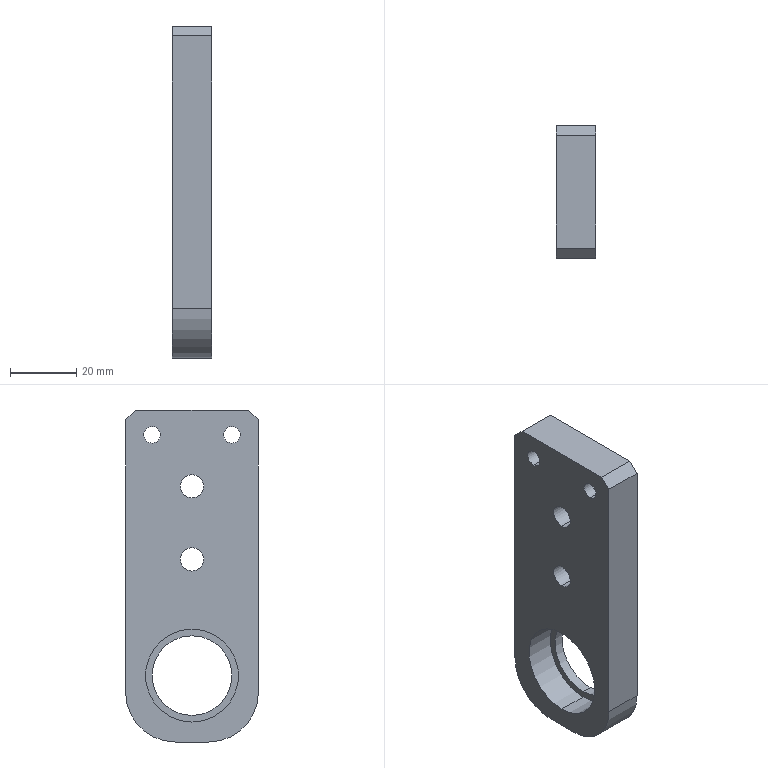Component | SolidWorks | ConveyorDrivenWheelSidePlate-4 | 1 solid | 23 faces | box 12 x 40 x 100 mm | volume 38439 mm3 | cylinder 14 | plane 9 | commonest cylinder face diameters 5 x4 7 x4 24 x2 28 x2 30 x2 | material Plain Carbon Steel
build123d program:
from build123d import *

# Parameters (mm, degrees)
SKETCH1_W           = 100
SKETCH1_H           = 40
BOSS_EXTRUDE1_DEPTH = 12
SKETCH2_R           = 14
CUT_EXTRUDE1_DEPTH  = 9
SKETCH3_R           = 3.5
CUT_EXTRUDE2_DEPTH  = 56.172
SKETCH4_R           = 12
CUT_EXTRUDE3_DEPTH  = 55.599
FILLET1_R           = 15
CHAMFER1_SIZE       = 3
M6_TAPPED_HOLE1_D   = 5


with BuildPart() as part:
    # Sketch1 → Boss-Extrude1 (new body)
    with BuildSketch(Plane(origin=(0, 0, 0), x_dir=(0, 0, -1), z_dir=(1, 0, 0))):
        Rectangle(SKETCH1_W, SKETCH1_H)
    extrude(amount=BOSS_EXTRUDE1_DEPTH)

    # Sketch2 → Cut-Extrude1 (cut)
    with BuildSketch(Plane(origin=(12, 0, 0), x_dir=(0, 0, -1), z_dir=(1, 0, 0))):
        with Locations((30, 0)):
            Circle(SKETCH2_R)
    extrude(amount=-CUT_EXTRUDE1_DEPTH, mode=Mode.SUBTRACT)

    # Sketch3 → Cut-Extrude2 (cut, through all)
    with BuildSketch(Plane.ZY):
        with Locations((5, 0)):
            Circle(SKETCH3_R)
        with Locations((27, 0)):
            Circle(SKETCH3_R)
    extrude(amount=-CUT_EXTRUDE2_DEPTH, mode=Mode.SUBTRACT)

    # Sketch4 → Cut-Extrude3 (cut, through all)
    with BuildSketch(Plane(origin=(3, 0, 0), x_dir=(0, 0, -1), z_dir=(1, 0, 0))):
        with Locations((30, 0)):
            Circle(SKETCH4_R)
    extrude(amount=-CUT_EXTRUDE3_DEPTH, mode=Mode.SUBTRACT)

    # Fillet1
    fillet1_edges = [part.edges().sort_by_distance(p)[0] for p in [
        (6, -20, -50),
        (6, 20, -50),
    ]]
    fillet(fillet1_edges, radius=FILLET1_R)

    # Chamfer1
    chamfer1_edges = [part.edges().sort_by_distance(p)[0] for p in [
        (6, -20, 50),
        (6, 20, 50),
    ]]
    chamfer(chamfer1_edges, length=CHAMFER1_SIZE)

    # M6 Tapped Hole1 (through all)
    with Locations(Plane.ZY):
        with Locations((42.5, 12), (42.5, -12)):
            Hole(M6_TAPPED_HOLE1_D / 2)


solid = part.part

# Placed as in the assembly
solid = solid.moved(Location((47.45, 5.646, 185), (0, 0, 180)))
STEP:
#1=COLOUR_RGB('',0.7922,0.8196,0.9333);
#2=FILL_AREA_STYLE_COLOUR('',#1);
#3=FILL_AREA_STYLE('',(#2));
#4=SURFACE_STYLE_FILL_AREA(#3);
#5=SURFACE_SIDE_STYLE('',(#4));
#6=SURFACE_STYLE_USAGE(.BOTH.,#5);
#7=PRESENTATION_STYLE_ASSIGNMENT((#6));
#8=CARTESIAN_POINT('',(1.396,-0.2502,8.858));
#9=VERTEX_POINT('',#8);
#10=CARTESIAN_POINT('',(1.396,-0.2502,9.055));
#11=VERTEX_POINT('',#10);
#12=CARTESIAN_POINT('',(1.396,-0.2502,8.957));
#13=DIRECTION('',(1.,-0.,-0.));
#14=DIRECTION('',(0.,0.,1.));
#15=AXIS2_PLACEMENT_3D('',#12,#13,#14);
#16=CIRCLE('',#15,0.09843);
#17=EDGE_CURVE('',#9,#11,#16,.T.);
#18=ORIENTED_EDGE('',*,*,#17,.F.);
#19=CARTESIAN_POINT('',(1.868,-0.2502,8.858));
#20=VERTEX_POINT('',#19);
#21=CARTESIAN_POINT('',(1.868,-0.2502,8.858));
#22=DIRECTION('',(1.,-0.,-0.));
#23=VECTOR('',#22,39.37);
#24=LINE('',#21,#23);
#25=EDGE_CURVE('',#9,#20,#24,.T.);
#26=ORIENTED_EDGE('',*,*,#25,.T.);
#27=CARTESIAN_POINT('',(1.868,-0.2502,9.055));
#28=VERTEX_POINT('',#27);
#29=CARTESIAN_POINT('',(1.868,-0.2502,8.957));
#30=DIRECTION('',(1.,-0.,-0.));
#31=DIRECTION('',(0.,0.,1.));
#32=AXIS2_PLACEMENT_3D('',#29,#30,#31);
#33=CIRCLE('',#32,0.09843);
#34=EDGE_CURVE('',#20,#28,#33,.T.);
#35=ORIENTED_EDGE('',*,*,#34,.T.);
#36=CARTESIAN_POINT('',(1.868,-0.2502,9.055));
#37=DIRECTION('',(1.,-0.,-0.));
#38=VECTOR('',#37,39.37);
#39=LINE('',#36,#38);
#40=EDGE_CURVE('',#11,#28,#39,.T.);
#41=ORIENTED_EDGE('',*,*,#40,.F.);
#42=EDGE_LOOP('',(#18,#26,#35,#41));
#43=FACE_OUTER_BOUND('',#42,.T.);
#44=CARTESIAN_POINT('',(1.868,-0.2502,8.957));
#45=DIRECTION('',(1.,-0.,-0.));
#46=DIRECTION('',(0.,0.,1.));
#47=AXIS2_PLACEMENT_3D('',#44,#45,#46);
#48=CYLINDRICAL_SURFACE('',#47,0.09843);
#49=ADVANCED_FACE('',(#43),#48,.F.);
#50=CARTESIAN_POINT('',(1.396,0.6947,8.858));
#51=VERTEX_POINT('',#50);
#52=CARTESIAN_POINT('',(1.396,0.6947,9.055));
#53=VERTEX_POINT('',#52);
#54=CARTESIAN_POINT('',(1.396,0.6947,8.957));
#55=DIRECTION('',(1.,-0.,-0.));
#56=DIRECTION('',(0.,0.,1.));
#57=AXIS2_PLACEMENT_3D('',#54,#55,#56);
#58=CIRCLE('',#57,0.09843);
#59=EDGE_CURVE('',#51,#53,#58,.T.);
#60=ORIENTED_EDGE('',*,*,#59,.F.);
#61=CARTESIAN_POINT('',(1.868,0.6947,8.858));
#62=VERTEX_POINT('',#61);
#63=CARTESIAN_POINT('',(1.868,0.6947,8.858));
#64=DIRECTION('',(1.,-0.,-0.));
#65=VECTOR('',#64,39.37);
#66=LINE('',#63,#65);
#67=EDGE_CURVE('',#51,#62,#66,.T.);
#68=ORIENTED_EDGE('',*,*,#67,.T.);
#69=CARTESIAN_POINT('',(1.868,0.6947,9.055));
#70=VERTEX_POINT('',#69);
#71=CARTESIAN_POINT('',(1.868,0.6947,8.957));
#72=DIRECTION('',(1.,-0.,-0.));
#73=DIRECTION('',(0.,0.,1.));
#74=AXIS2_PLACEMENT_3D('',#71,#72,#73);
#75=CIRCLE('',#74,0.09843);
#76=EDGE_CURVE('',#62,#70,#75,.T.);
#77=ORIENTED_EDGE('',*,*,#76,.T.);
#78=CARTESIAN_POINT('',(1.868,0.6947,9.055));
#79=DIRECTION('',(1.,-0.,-0.));
#80=VECTOR('',#79,39.37);
#81=LINE('',#78,#80);
#82=EDGE_CURVE('',#53,#70,#81,.T.);
#83=ORIENTED_EDGE('',*,*,#82,.F.);
#84=EDGE_LOOP('',(#60,#68,#77,#83));
#85=FACE_OUTER_BOUND('',#84,.T.);
#86=CARTESIAN_POINT('',(1.868,0.6947,8.957));
#87=DIRECTION('',(1.,-0.,-0.));
#88=DIRECTION('',(0.,0.,1.));
#89=AXIS2_PLACEMENT_3D('',#86,#87,#88);
#90=CYLINDRICAL_SURFACE('',#89,0.09843);
#91=ADVANCED_FACE('',(#85),#90,.F.);
#92=CARTESIAN_POINT('',(1.868,0.2223,6.575));
#93=VERTEX_POINT('',#92);
#94=CARTESIAN_POINT('',(1.868,0.2223,5.63));
#95=VERTEX_POINT('',#94);
#96=CARTESIAN_POINT('',(1.868,0.2223,6.102));
#97=DIRECTION('',(-1.,0.,0.));
#98=DIRECTION('',(0.,0.,-1.));
#99=AXIS2_PLACEMENT_3D('',#96,#97,#98);
#100=CIRCLE('',#99,0.4724);
#101=EDGE_CURVE('',#93,#95,#100,.T.);
#102=ORIENTED_EDGE('',*,*,#101,.F.);
#103=CARTESIAN_POINT('',(1.75,0.2223,6.575));
#104=VERTEX_POINT('',#103);
#105=CARTESIAN_POINT('',(1.868,0.2223,6.575));
#106=DIRECTION('',(-1.,0.,0.));
#107=VECTOR('',#106,39.37);
#108=LINE('',#105,#107);
#109=EDGE_CURVE('',#93,#104,#108,.T.);
#110=ORIENTED_EDGE('',*,*,#109,.T.);
#111=CARTESIAN_POINT('',(1.75,0.2223,5.63));
#112=VERTEX_POINT('',#111);
#113=CARTESIAN_POINT('',(1.75,0.2223,6.102));
#114=DIRECTION('',(-1.,0.,0.));
#115=DIRECTION('',(0.,0.,-1.));
#116=AXIS2_PLACEMENT_3D('',#113,#114,#115);
#117=CIRCLE('',#116,0.4724);
#118=EDGE_CURVE('',#104,#112,#117,.T.);
#119=ORIENTED_EDGE('',*,*,#118,.T.);
#120=CARTESIAN_POINT('',(1.868,0.2223,5.63));
#121=DIRECTION('',(-1.,0.,0.));
#122=VECTOR('',#121,39.37);
#123=LINE('',#120,#122);
#124=EDGE_CURVE('',#95,#112,#123,.T.);
#125=ORIENTED_EDGE('',*,*,#124,.F.);
#126=EDGE_LOOP('',(#102,#110,#119,#125));
#127=FACE_OUTER_BOUND('',#126,.T.);
#128=CARTESIAN_POINT('',(1.868,0.2223,6.102));
#129=DIRECTION('',(-1.,0.,0.));
#130=DIRECTION('',(0.,0.,-1.));
#131=AXIS2_PLACEMENT_3D('',#128,#129,#130);
#132=CYLINDRICAL_SURFACE('',#131,0.4724);
#133=ADVANCED_FACE('',(#127),#132,.F.);
#134=CARTESIAN_POINT('',(1.396,0.2223,8.209));
#135=VERTEX_POINT('',#134);
#136=CARTESIAN_POINT('',(1.396,0.2223,8.484));
#137=VERTEX_POINT('',#136);
#138=CARTESIAN_POINT('',(1.396,0.2223,8.346));
#139=DIRECTION('',(1.,-0.,-0.));
#140=DIRECTION('',(0.,0.,1.));
#141=AXIS2_PLACEMENT_3D('',#138,#139,#140);
#142=CIRCLE('',#141,0.1378);
#143=EDGE_CURVE('',#135,#137,#142,.T.);
#144=ORIENTED_EDGE('',*,*,#143,.F.);
#145=CARTESIAN_POINT('',(1.868,0.2223,8.209));
#146=VERTEX_POINT('',#145);
#147=CARTESIAN_POINT('',(1.396,0.2223,8.209));
#148=DIRECTION('',(1.,-0.,-0.));
#149=VECTOR('',#148,39.37);
#150=LINE('',#147,#149);
#151=EDGE_CURVE('',#135,#146,#150,.T.);
#152=ORIENTED_EDGE('',*,*,#151,.T.);
#153=CARTESIAN_POINT('',(1.868,0.2223,8.484));
#154=VERTEX_POINT('',#153);
#155=CARTESIAN_POINT('',(1.868,0.2223,8.346));
#156=DIRECTION('',(1.,-0.,-0.));
#157=DIRECTION('',(0.,0.,1.));
#158=AXIS2_PLACEMENT_3D('',#155,#156,#157);
#159=CIRCLE('',#158,0.1378);
#160=EDGE_CURVE('',#146,#154,#159,.T.);
#161=ORIENTED_EDGE('',*,*,#160,.T.);
#162=CARTESIAN_POINT('',(1.396,0.2223,8.484));
#163=DIRECTION('',(1.,-0.,-0.));
#164=VECTOR('',#163,39.37);
#165=LINE('',#162,#164);
#166=EDGE_CURVE('',#137,#154,#165,.T.);
#167=ORIENTED_EDGE('',*,*,#166,.F.);
#168=EDGE_LOOP('',(#144,#152,#161,#167));
#169=FACE_OUTER_BOUND('',#168,.T.);
#170=CARTESIAN_POINT('',(1.396,0.2223,8.346));
#171=DIRECTION('',(1.,-0.,-0.));
#172=DIRECTION('',(0.,0.,1.));
#173=AXIS2_PLACEMENT_3D('',#170,#171,#172);
#174=CYLINDRICAL_SURFACE('',#173,0.1378);
#175=ADVANCED_FACE('',(#169),#174,.F.);
#176=CARTESIAN_POINT('',(1.396,0.2223,7.343));
#177=VERTEX_POINT('',#176);
#178=CARTESIAN_POINT('',(1.396,0.2223,7.618));
#179=VERTEX_POINT('',#178);
#180=CARTESIAN_POINT('',(1.396,0.2223,7.48));
#181=DIRECTION('',(1.,-0.,-0.));
#182=DIRECTION('',(0.,0.,1.));
#183=AXIS2_PLACEMENT_3D('',#180,#181,#182);
#184=CIRCLE('',#183,0.1378);
#185=EDGE_CURVE('',#177,#179,#184,.T.);
#186=ORIENTED_EDGE('',*,*,#185,.F.);
#187=CARTESIAN_POINT('',(1.868,0.2223,7.343));
#188=VERTEX_POINT('',#187);
#189=CARTESIAN_POINT('',(1.396,0.2223,7.343));
#190=DIRECTION('',(1.,-0.,-0.));
#191=VECTOR('',#190,39.37);
#192=LINE('',#189,#191);
#193=EDGE_CURVE('',#177,#188,#192,.T.);
#194=ORIENTED_EDGE('',*,*,#193,.T.);
#195=CARTESIAN_POINT('',(1.868,0.2223,7.618));
#196=VERTEX_POINT('',#195);
#197=CARTESIAN_POINT('',(1.868,0.2223,7.48));
#198=DIRECTION('',(1.,-0.,-0.));
#199=DIRECTION('',(0.,0.,1.));
#200=AXIS2_PLACEMENT_3D('',#197,#198,#199);
#201=CIRCLE('',#200,0.1378);
#202=EDGE_CURVE('',#188,#196,#201,.T.);
#203=ORIENTED_EDGE('',*,*,#202,.T.);
#204=CARTESIAN_POINT('',(1.396,0.2223,7.618));
#205=DIRECTION('',(1.,-0.,-0.));
#206=VECTOR('',#205,39.37);
#207=LINE('',#204,#206);
#208=EDGE_CURVE('',#179,#196,#207,.T.);
#209=ORIENTED_EDGE('',*,*,#208,.F.);
#210=EDGE_LOOP('',(#186,#194,#203,#209));
#211=FACE_OUTER_BOUND('',#210,.T.);
#212=CARTESIAN_POINT('',(1.396,0.2223,7.48));
#213=DIRECTION('',(1.,-0.,-0.));
#214=DIRECTION('',(0.,0.,1.));
#215=AXIS2_PLACEMENT_3D('',#212,#213,#214);
#216=CYLINDRICAL_SURFACE('',#215,0.1378);
#217=ADVANCED_FACE('',(#211),#216,.F.);
#218=CARTESIAN_POINT('',(1.75,0.2223,6.654));
#219=VERTEX_POINT('',#218);
#220=CARTESIAN_POINT('',(1.75,0.2223,5.551));
#221=VERTEX_POINT('',#220);
#222=CARTESIAN_POINT('',(1.75,0.2223,6.102));
#223=DIRECTION('',(-1.,0.,0.));
#224=DIRECTION('',(0.,0.,-1.));
#225=AXIS2_PLACEMENT_3D('',#222,#223,#224);
#226=CIRCLE('',#225,0.5512);
#227=EDGE_CURVE('',#219,#221,#226,.T.);
#228=ORIENTED_EDGE('',*,*,#227,.F.);
#229=CARTESIAN_POINT('',(1.396,0.2223,6.654));
#230=VERTEX_POINT('',#229);
#231=CARTESIAN_POINT('',(1.75,0.2223,6.654));
#232=DIRECTION('',(-1.,0.,0.));
#233=VECTOR('',#232,39.37);
#234=LINE('',#231,#233);
#235=EDGE_CURVE('',#219,#230,#234,.T.);
#236=ORIENTED_EDGE('',*,*,#235,.T.);
#237=CARTESIAN_POINT('',(1.396,0.2223,5.551));
#238=VERTEX_POINT('',#237);
#239=CARTESIAN_POINT('',(1.396,0.2223,6.102));
#240=DIRECTION('',(-1.,0.,0.));
#241=DIRECTION('',(0.,0.,-1.));
#242=AXIS2_PLACEMENT_3D('',#239,#240,#241);
#243=CIRCLE('',#242,0.5512);
#244=EDGE_CURVE('',#230,#238,#243,.T.);
#245=ORIENTED_EDGE('',*,*,#244,.T.);
#246=CARTESIAN_POINT('',(1.75,0.2223,5.551));
#247=DIRECTION('',(-1.,0.,0.));
#248=VECTOR('',#247,39.37);
#249=LINE('',#246,#248);
#250=EDGE_CURVE('',#221,#238,#249,.T.);
#251=ORIENTED_EDGE('',*,*,#250,.F.);
#252=EDGE_LOOP('',(#228,#236,#245,#251));
#253=FACE_OUTER_BOUND('',#252,.T.);
#254=CARTESIAN_POINT('',(1.75,0.2223,6.102));
#255=DIRECTION('',(-1.,0.,0.));
#256=DIRECTION('',(0.,0.,-1.));
#257=AXIS2_PLACEMENT_3D('',#254,#255,#256);
#258=CYLINDRICAL_SURFACE('',#257,0.5512);
#259=ADVANCED_FACE('',(#253),#258,.F.);
#260=CARTESIAN_POINT('',(1.396,0.4191,5.315));
#261=VERTEX_POINT('',#260);
#262=CARTESIAN_POINT('',(1.396,0.02542,5.315));
#263=VERTEX_POINT('',#262);
#264=CARTESIAN_POINT('',(1.396,1.01,5.315));
#265=DIRECTION('',(-0.,-1.,0.));
#266=VECTOR('',#265,39.37);
#267=LINE('',#264,#266);
#268=EDGE_CURVE('',#261,#263,#267,.T.);
#269=ORIENTED_EDGE('',*,*,#268,.F.);
#270=CARTESIAN_POINT('',(1.868,0.4191,5.315));
#271=VERTEX_POINT('',#270);
#272=CARTESIAN_POINT('',(1.396,0.4191,5.315));
#273=DIRECTION('',(1.,-0.,-0.));
#274=VECTOR('',#273,39.37);
#275=LINE('',#272,#274);
#276=EDGE_CURVE('',#261,#271,#275,.T.);
#277=ORIENTED_EDGE('',*,*,#276,.T.);
#278=CARTESIAN_POINT('',(1.868,0.02542,5.315));
#279=VERTEX_POINT('',#278);
#280=CARTESIAN_POINT('',(1.868,1.01,5.315));
#281=DIRECTION('',(-0.,-1.,0.));
#282=VECTOR('',#281,39.37);
#283=LINE('',#280,#282);
#284=EDGE_CURVE('',#271,#279,#283,.T.);
#285=ORIENTED_EDGE('',*,*,#284,.T.);
#286=CARTESIAN_POINT('',(1.396,0.02542,5.315));
#287=DIRECTION('',(-1.,0.,0.));
#288=VECTOR('',#287,39.37);
#289=LINE('',#286,#288);
#290=EDGE_CURVE('',#279,#263,#289,.T.);
#291=ORIENTED_EDGE('',*,*,#290,.T.);
#292=EDGE_LOOP('',(#269,#277,#285,#291));
#293=FACE_OUTER_BOUND('',#292,.T.);
#294=CARTESIAN_POINT('',(1.396,1.01,5.315));
#295=DIRECTION('',(0.,-0.,1.));
#296=DIRECTION('',(-1.,0.,0.));
#297=AXIS2_PLACEMENT_3D('',#294,#295,#296);
#298=PLANE('',#297);
#299=ADVANCED_FACE('',(#293),#298,.F.);
#300=CARTESIAN_POINT('',(1.868,-0.5651,5.906));
#301=VERTEX_POINT('',#300);
#302=CARTESIAN_POINT('',(1.868,-0.5651,9.134));
#303=VERTEX_POINT('',#302);
#304=CARTESIAN_POINT('',(1.868,-0.5651,9.252));
#305=DIRECTION('',(0.,0.,1.));
#306=VECTOR('',#305,39.37);
#307=LINE('',#304,#306);
#308=EDGE_CURVE('',#301,#303,#307,.T.);
#309=ORIENTED_EDGE('',*,*,#308,.T.);
#310=CARTESIAN_POINT('',(1.396,-0.5651,9.134));
#311=VERTEX_POINT('',#310);
#312=CARTESIAN_POINT('',(1.396,-0.5651,9.134));
#313=DIRECTION('',(-1.,0.,0.));
#314=VECTOR('',#313,39.37);
#315=LINE('',#312,#314);
#316=EDGE_CURVE('',#303,#311,#315,.T.);
#317=ORIENTED_EDGE('',*,*,#316,.T.);
#318=CARTESIAN_POINT('',(1.396,-0.5651,5.906));
#319=VERTEX_POINT('',#318);
#320=CARTESIAN_POINT('',(1.396,-0.5651,9.252));
#321=DIRECTION('',(0.,0.,1.));
#322=VECTOR('',#321,39.37);
#323=LINE('',#320,#322);
#324=EDGE_CURVE('',#319,#311,#323,.T.);
#325=ORIENTED_EDGE('',*,*,#324,.F.);
#326=CARTESIAN_POINT('',(1.396,-0.5651,5.906));
#327=DIRECTION('',(1.,-0.,-0.));
#328=VECTOR('',#327,39.37);
#329=LINE('',#326,#328);
#330=EDGE_CURVE('',#319,#301,#329,.T.);
#331=ORIENTED_EDGE('',*,*,#330,.T.);
#332=EDGE_LOOP('',(#309,#317,#325,#331));
#333=FACE_OUTER_BOUND('',#332,.T.);
#334=CARTESIAN_POINT('',(1.396,-0.5651,9.252));
#335=DIRECTION('',(0.,1.,-0.));
#336=DIRECTION('',(-0.,0.,-1.));
#337=AXIS2_PLACEMENT_3D('',#334,#335,#336);
#338=PLANE('',#337);
#339=ADVANCED_FACE('',(#333),#338,.F.);
#340=CARTESIAN_POINT('',(1.868,-0.447,9.252));
#341=VERTEX_POINT('',#340);
#342=CARTESIAN_POINT('',(1.868,0.8916,9.252));
#343=VERTEX_POINT('',#342);
#344=CARTESIAN_POINT('',(1.868,1.01,9.252));
#345=DIRECTION('',(0.,1.,0.));
#346=VECTOR('',#345,39.37);
#347=LINE('',#344,#346);
#348=EDGE_CURVE('',#341,#343,#347,.T.);
#349=ORIENTED_EDGE('',*,*,#348,.T.);
#350=CARTESIAN_POINT('',(1.396,0.8916,9.252));
#351=VERTEX_POINT('',#350);
#352=CARTESIAN_POINT('',(1.396,0.8916,9.252));
#353=DIRECTION('',(-1.,0.,0.));
#354=VECTOR('',#353,39.37);
#355=LINE('',#352,#354);
#356=EDGE_CURVE('',#343,#351,#355,.T.);
#357=ORIENTED_EDGE('',*,*,#356,.T.);
#358=CARTESIAN_POINT('',(1.396,-0.447,9.252));
#359=VERTEX_POINT('',#358);
#360=CARTESIAN_POINT('',(1.396,1.01,9.252));
#361=DIRECTION('',(0.,1.,0.));
#362=VECTOR('',#361,39.37);
#363=LINE('',#360,#362);
#364=EDGE_CURVE('',#359,#351,#363,.T.);
#365=ORIENTED_EDGE('',*,*,#364,.F.);
#366=CARTESIAN_POINT('',(1.396,-0.447,9.252));
#367=DIRECTION('',(1.,-0.,-0.));
#368=VECTOR('',#367,39.37);
#369=LINE('',#366,#368);
#370=EDGE_CURVE('',#359,#341,#369,.T.);
#371=ORIENTED_EDGE('',*,*,#370,.T.);
#372=EDGE_LOOP('',(#349,#357,#365,#371));
#373=FACE_OUTER_BOUND('',#372,.T.);
#374=CARTESIAN_POINT('',(1.396,1.01,9.252));
#375=DIRECTION('',(-0.,0.,-1.));
#376=DIRECTION('',(1.,-0.,-0.));
#377=AXIS2_PLACEMENT_3D('',#374,#375,#376);
#378=PLANE('',#377);
#379=ADVANCED_FACE('',(#373),#378,.F.);
#380=CARTESIAN_POINT('',(1.396,1.01,9.134));
#381=VERTEX_POINT('',#380);
#382=CARTESIAN_POINT('',(1.396,1.01,5.906));
#383=VERTEX_POINT('',#382);
#384=CARTESIAN_POINT('',(1.396,1.01,9.252));
#385=DIRECTION('',(-0.,0.,-1.));
#386=VECTOR('',#385,39.37);
#387=LINE('',#384,#386);
#388=EDGE_CURVE('',#381,#383,#387,.T.);
#389=ORIENTED_EDGE('',*,*,#388,.F.);
#390=CARTESIAN_POINT('',(1.868,1.01,9.134));
#391=VERTEX_POINT('',#390);
#392=CARTESIAN_POINT('',(1.396,1.01,9.134));
#393=DIRECTION('',(1.,-0.,-0.));
#394=VECTOR('',#393,39.37);
#395=LINE('',#392,#394);
#396=EDGE_CURVE('',#381,#391,#395,.T.);
#397=ORIENTED_EDGE('',*,*,#396,.T.);
#398=CARTESIAN_POINT('',(1.868,1.01,5.906));
#399=VERTEX_POINT('',#398);
#400=CARTESIAN_POINT('',(1.868,1.01,9.252));
#401=DIRECTION('',(-0.,0.,-1.));
#402=VECTOR('',#401,39.37);
#403=LINE('',#400,#402);
#404=EDGE_CURVE('',#391,#399,#403,.T.);
#405=ORIENTED_EDGE('',*,*,#404,.T.);
#406=CARTESIAN_POINT('',(1.396,1.01,5.906));
#407=DIRECTION('',(-1.,0.,0.));
#408=VECTOR('',#407,39.37);
#409=LINE('',#406,#408);
#410=EDGE_CURVE('',#399,#383,#409,.T.);
#411=ORIENTED_EDGE('',*,*,#410,.T.);
#412=EDGE_LOOP('',(#389,#397,#405,#411));
#413=FACE_OUTER_BOUND('',#412,.T.);
#414=CARTESIAN_POINT('',(1.396,1.01,9.252));
#415=DIRECTION('',(-0.,-1.,0.));
#416=DIRECTION('',(0.,0.,1.));
#417=AXIS2_PLACEMENT_3D('',#414,#415,#416);
#418=PLANE('',#417);
#419=ADVANCED_FACE('',(#413),#418,.F.);
#420=CARTESIAN_POINT('',(1.396,-0.2502,8.957));
#421=DIRECTION('',(1.,-0.,-0.));
#422=DIRECTION('',(0.,0.,1.));
#423=AXIS2_PLACEMENT_3D('',#420,#421,#422);
#424=CIRCLE('',#423,0.09843);
#425=EDGE_CURVE('',#11,#9,#424,.T.);
#426=ORIENTED_EDGE('',*,*,#425,.T.);
#427=ORIENTED_EDGE('',*,*,#17,.T.);
#428=EDGE_LOOP('',(#426,#427));
#429=FACE_BOUND('',#428,.T.);
#430=CARTESIAN_POINT('',(1.396,0.6947,8.957));
#431=DIRECTION('',(1.,-0.,-0.));
#432=DIRECTION('',(0.,0.,1.));
#433=AXIS2_PLACEMENT_3D('',#430,#431,#432);
#434=CIRCLE('',#433,0.09843);
#435=EDGE_CURVE('',#53,#51,#434,.T.);
#436=ORIENTED_EDGE('',*,*,#435,.T.);
#437=ORIENTED_EDGE('',*,*,#59,.T.);
#438=EDGE_LOOP('',(#436,#437));
#439=FACE_BOUND('',#438,.T.);
#440=CARTESIAN_POINT('',(1.396,0.2223,8.346));
#441=DIRECTION('',(1.,-0.,-0.));
#442=DIRECTION('',(0.,0.,1.));
#443=AXIS2_PLACEMENT_3D('',#440,#441,#442);
#444=CIRCLE('',#443,0.1378);
#445=EDGE_CURVE('',#137,#135,#444,.T.);
#446=ORIENTED_EDGE('',*,*,#445,.T.);
#447=ORIENTED_EDGE('',*,*,#143,.T.);
#448=EDGE_LOOP('',(#446,#447));
#449=FACE_BOUND('',#448,.T.);
#450=CARTESIAN_POINT('',(1.396,0.2223,7.48));
#451=DIRECTION('',(1.,-0.,-0.));
#452=DIRECTION('',(0.,0.,1.));
#453=AXIS2_PLACEMENT_3D('',#450,#451,#452);
#454=CIRCLE('',#453,0.1378);
#455=EDGE_CURVE('',#179,#177,#454,.T.);
#456=ORIENTED_EDGE('',*,*,#455,.T.);
#457=ORIENTED_EDGE('',*,*,#185,.T.);
#458=EDGE_LOOP('',(#456,#457));
#459=FACE_BOUND('',#458,.T.);
#460=CARTESIAN_POINT('',(1.396,0.2223,6.102));
#461=DIRECTION('',(-1.,0.,0.));
#462=DIRECTION('',(0.,0.,-1.));
#463=AXIS2_PLACEMENT_3D('',#460,#461,#462);
#464=CIRCLE('',#463,0.5512);
#465=EDGE_CURVE('',#238,#230,#464,.T.);
#466=ORIENTED_EDGE('',*,*,#465,.F.);
#467=ORIENTED_EDGE('',*,*,#244,.F.);
#468=EDGE_LOOP('',(#466,#467));
#469=FACE_BOUND('',#468,.T.);
#470=ORIENTED_EDGE('',*,*,#364,.T.);
#471=CARTESIAN_POINT('',(1.396,1.01,9.134));
#472=DIRECTION('',(0.,0.7071,-0.7071));
#473=VECTOR('',#472,39.37);
#474=LINE('',#471,#473);
#475=EDGE_CURVE('',#351,#381,#474,.T.);
#476=ORIENTED_EDGE('',*,*,#475,.T.);
#477=ORIENTED_EDGE('',*,*,#388,.T.);
#478=CARTESIAN_POINT('',(1.396,0.4191,5.906));
#479=DIRECTION('',(-1.,0.,0.));
#480=DIRECTION('',(0.,0.,1.));
#481=AXIS2_PLACEMENT_3D('',#478,#479,#480);
#482=CIRCLE('',#481,0.5906);
#483=EDGE_CURVE('',#383,#261,#482,.T.);
#484=ORIENTED_EDGE('',*,*,#483,.T.);
#485=ORIENTED_EDGE('',*,*,#268,.T.);
#486=CARTESIAN_POINT('',(1.396,0.02542,5.906));
#487=DIRECTION('',(-1.,0.,0.));
#488=DIRECTION('',(0.,0.,1.));
#489=AXIS2_PLACEMENT_3D('',#486,#487,#488);
#490=CIRCLE('',#489,0.5906);
#491=EDGE_CURVE('',#263,#319,#490,.T.);
#492=ORIENTED_EDGE('',*,*,#491,.T.);
#493=ORIENTED_EDGE('',*,*,#324,.T.);
#494=CARTESIAN_POINT('',(1.396,-0.447,9.252));
#495=DIRECTION('',(0.,0.7071,0.7071));
#496=VECTOR('',#495,39.37);
#497=LINE('',#494,#496);
#498=EDGE_CURVE('',#311,#359,#497,.T.);
#499=ORIENTED_EDGE('',*,*,#498,.T.);
#500=EDGE_LOOP('',(#470,#476,#477,#484,#485,#492,#493,#499));
#501=FACE_OUTER_BOUND('',#500,.T.);
#502=CARTESIAN_POINT('',(1.396,0.2223,7.283));
#503=DIRECTION('',(1.,-0.,-0.));
#504=DIRECTION('',(0.,0.,1.));
#505=AXIS2_PLACEMENT_3D('',#502,#503,#504);
#506=PLANE('',#505);
#507=ADVANCED_FACE('',(#429,#439,#449,#459,#469,#501),#506,.F.);
#508=CARTESIAN_POINT('',(1.868,-0.2502,8.957));
#509=DIRECTION('',(1.,-0.,-0.));
#510=DIRECTION('',(0.,0.,1.));
#511=AXIS2_PLACEMENT_3D('',#508,#509,#510);
#512=CIRCLE('',#511,0.09843);
#513=EDGE_CURVE('',#28,#20,#512,.T.);
#514=ORIENTED_EDGE('',*,*,#513,.F.);
#515=ORIENTED_EDGE('',*,*,#34,.F.);
#516=EDGE_LOOP('',(#514,#515));
#517=FACE_BOUND('',#516,.T.);
#518=CARTESIAN_POINT('',(1.868,0.6947,8.957));
#519=DIRECTION('',(1.,-0.,-0.));
#520=DIRECTION('',(0.,0.,1.));
#521=AXIS2_PLACEMENT_3D('',#518,#519,#520);
#522=CIRCLE('',#521,0.09843);
#523=EDGE_CURVE('',#70,#62,#522,.T.);
#524=ORIENTED_EDGE('',*,*,#523,.F.);
#525=ORIENTED_EDGE('',*,*,#76,.F.);
#526=EDGE_LOOP('',(#524,#525));
#527=FACE_BOUND('',#526,.T.);
#528=CARTESIAN_POINT('',(1.868,0.2223,6.102));
#529=DIRECTION('',(-1.,0.,0.));
#530=DIRECTION('',(0.,0.,-1.));
#531=AXIS2_PLACEMENT_3D('',#528,#529,#530);
#532=CIRCLE('',#531,0.4724);
#533=EDGE_CURVE('',#95,#93,#532,.T.);
#534=ORIENTED_EDGE('',*,*,#533,.T.);
#535=ORIENTED_EDGE('',*,*,#101,.T.);
#536=EDGE_LOOP('',(#534,#535));
#537=FACE_BOUND('',#536,.T.);
#538=CARTESIAN_POINT('',(1.868,0.2223,8.346));
#539=DIRECTION('',(1.,-0.,-0.));
#540=DIRECTION('',(0.,0.,1.));
#541=AXIS2_PLACEMENT_3D('',#538,#539,#540);
#542=CIRCLE('',#541,0.1378);
#543=EDGE_CURVE('',#154,#146,#542,.T.);
#544=ORIENTED_EDGE('',*,*,#543,.F.);
#545=ORIENTED_EDGE('',*,*,#160,.F.);
#546=EDGE_LOOP('',(#544,#545));
#547=FACE_BOUND('',#546,.T.);
#548=CARTESIAN_POINT('',(1.868,0.2223,7.48));
#549=DIRECTION('',(1.,-0.,-0.));
#550=DIRECTION('',(0.,0.,1.));
#551=AXIS2_PLACEMENT_3D('',#548,#549,#550);
#552=CIRCLE('',#551,0.1378);
#553=EDGE_CURVE('',#196,#188,#552,.T.);
#554=ORIENTED_EDGE('',*,*,#553,.F.);
#555=ORIENTED_EDGE('',*,*,#202,.F.);
#556=EDGE_LOOP('',(#554,#555));
#557=FACE_BOUND('',#556,.T.);
#558=ORIENTED_EDGE('',*,*,#404,.F.);
#559=CARTESIAN_POINT('',(1.868,1.541,8.602));
#560=DIRECTION('',(-0.,-0.7071,0.7071));
#561=VECTOR('',#560,39.37);
#562=LINE('',#559,#561);
#563=EDGE_CURVE('',#391,#343,#562,.T.);
#564=ORIENTED_EDGE('',*,*,#563,.T.);
#565=ORIENTED_EDGE('',*,*,#348,.F.);
#566=CARTESIAN_POINT('',(1.868,-1.097,8.602));
#567=DIRECTION('',(-0.,-0.7071,-0.7071));
#568=VECTOR('',#567,39.37);
#569=LINE('',#566,#568);
#570=EDGE_CURVE('',#341,#303,#569,.T.);
#571=ORIENTED_EDGE('',*,*,#570,.T.);
#572=ORIENTED_EDGE('',*,*,#308,.F.);
#573=CARTESIAN_POINT('',(1.868,0.02542,5.906));
#574=DIRECTION('',(1.,-0.,-0.));
#575=DIRECTION('',(0.,0.,1.));
#576=AXIS2_PLACEMENT_3D('',#573,#574,#575);
#577=CIRCLE('',#576,0.5906);
#578=EDGE_CURVE('',#301,#279,#577,.T.);
#579=ORIENTED_EDGE('',*,*,#578,.T.);
#580=ORIENTED_EDGE('',*,*,#284,.F.);
#581=CARTESIAN_POINT('',(1.868,0.4191,5.906));
#582=DIRECTION('',(1.,-0.,-0.));
#583=DIRECTION('',(0.,0.,1.));
#584=AXIS2_PLACEMENT_3D('',#581,#582,#583);
#585=CIRCLE('',#584,0.5906);
#586=EDGE_CURVE('',#271,#399,#585,.T.);
#587=ORIENTED_EDGE('',*,*,#586,.T.);
#588=EDGE_LOOP('',(#558,#564,#565,#571,#572,#579,#580,#587));
#589=FACE_OUTER_BOUND('',#588,.T.);
#590=CARTESIAN_POINT('',(1.868,0.2223,7.283));
#591=DIRECTION('',(1.,-0.,-0.));
#592=DIRECTION('',(0.,0.,1.));
#593=AXIS2_PLACEMENT_3D('',#590,#591,#592);
#594=PLANE('',#593);
#595=ADVANCED_FACE('',(#517,#527,#537,#547,#557,#589),#594,.T.);
#596=ORIENTED_EDGE('',*,*,#235,.F.);
#597=CARTESIAN_POINT('',(1.75,0.2223,6.102));
#598=DIRECTION('',(-1.,0.,0.));
#599=DIRECTION('',(0.,0.,-1.));
#600=AXIS2_PLACEMENT_3D('',#597,#598,#599);
#601=CIRCLE('',#600,0.5512);
#602=EDGE_CURVE('',#221,#219,#601,.T.);
#603=ORIENTED_EDGE('',*,*,#602,.F.);
#604=ORIENTED_EDGE('',*,*,#250,.T.);
#605=ORIENTED_EDGE('',*,*,#465,.T.);
#606=EDGE_LOOP('',(#596,#603,#604,#605));
#607=FACE_OUTER_BOUND('',#606,.T.);
#608=CARTESIAN_POINT('',(1.75,0.2223,6.102));
#609=DIRECTION('',(-1.,0.,0.));
#610=DIRECTION('',(0.,0.,-1.));
#611=AXIS2_PLACEMENT_3D('',#608,#609,#610);
#612=CYLINDRICAL_SURFACE('',#611,0.5512);
#613=ADVANCED_FACE('',(#607),#612,.F.);
#614=CARTESIAN_POINT('',(1.75,0.2223,6.102));
#615=DIRECTION('',(-1.,0.,0.));
#616=DIRECTION('',(0.,0.,-1.));
#617=AXIS2_PLACEMENT_3D('',#614,#615,#616);
#618=CIRCLE('',#617,0.4724);
#619=EDGE_CURVE('',#112,#104,#618,.T.);
#620=ORIENTED_EDGE('',*,*,#619,.F.);
#621=ORIENTED_EDGE('',*,*,#118,.F.);
#622=EDGE_LOOP('',(#620,#621));
#623=FACE_BOUND('',#622,.T.);
#624=ORIENTED_EDGE('',*,*,#602,.T.);
#625=ORIENTED_EDGE('',*,*,#227,.T.);
#626=EDGE_LOOP('',(#624,#625));
#627=FACE_OUTER_BOUND('',#626,.T.);
#628=CARTESIAN_POINT('',(1.75,0.2223,6.102));
#629=DIRECTION('',(-1.,0.,0.));
#630=DIRECTION('',(-0.,0.,-1.));
#631=AXIS2_PLACEMENT_3D('',#628,#629,#630);
#632=PLANE('',#631);
#633=ADVANCED_FACE('',(#623,#627),#632,.T.);
#634=ORIENTED_EDGE('',*,*,#193,.F.);
#635=ORIENTED_EDGE('',*,*,#455,.F.);
#636=ORIENTED_EDGE('',*,*,#208,.T.);
#637=ORIENTED_EDGE('',*,*,#553,.T.);
#638=EDGE_LOOP('',(#634,#635,#636,#637));
#639=FACE_OUTER_BOUND('',#638,.T.);
#640=CARTESIAN_POINT('',(1.396,0.2223,7.48));
#641=DIRECTION('',(1.,-0.,-0.));
#642=DIRECTION('',(0.,0.,1.));
#643=AXIS2_PLACEMENT_3D('',#640,#641,#642);
#644=CYLINDRICAL_SURFACE('',#643,0.1378);
#645=ADVANCED_FACE('',(#639),#644,.F.);
#646=ORIENTED_EDGE('',*,*,#151,.F.);
#647=ORIENTED_EDGE('',*,*,#445,.F.);
#648=ORIENTED_EDGE('',*,*,#166,.T.);
#649=ORIENTED_EDGE('',*,*,#543,.T.);
#650=EDGE_LOOP('',(#646,#647,#648,#649));
#651=FACE_OUTER_BOUND('',#650,.T.);
#652=CARTESIAN_POINT('',(1.396,0.2223,8.346));
#653=DIRECTION('',(1.,-0.,-0.));
#654=DIRECTION('',(0.,0.,1.));
#655=AXIS2_PLACEMENT_3D('',#652,#653,#654);
#656=CYLINDRICAL_SURFACE('',#655,0.1378);
#657=ADVANCED_FACE('',(#651),#656,.F.);
#658=ORIENTED_EDGE('',*,*,#109,.F.);
#659=ORIENTED_EDGE('',*,*,#533,.F.);
#660=ORIENTED_EDGE('',*,*,#124,.T.);
#661=ORIENTED_EDGE('',*,*,#619,.T.);
#662=EDGE_LOOP('',(#658,#659,#660,#661));
#663=FACE_OUTER_BOUND('',#662,.T.);
#664=CARTESIAN_POINT('',(1.868,0.2223,6.102));
#665=DIRECTION('',(-1.,0.,0.));
#666=DIRECTION('',(0.,0.,-1.));
#667=AXIS2_PLACEMENT_3D('',#664,#665,#666);
#668=CYLINDRICAL_SURFACE('',#667,0.4724);
#669=ADVANCED_FACE('',(#663),#668,.F.);
#670=ORIENTED_EDGE('',*,*,#483,.F.);
#671=ORIENTED_EDGE('',*,*,#410,.F.);
#672=ORIENTED_EDGE('',*,*,#586,.F.);
#673=ORIENTED_EDGE('',*,*,#276,.F.);
#674=EDGE_LOOP('',(#670,#671,#672,#673));
#675=FACE_OUTER_BOUND('',#674,.T.);
#676=CARTESIAN_POINT('',(1.396,0.4191,5.906));
#677=DIRECTION('',(1.,-0.,-0.));
#678=DIRECTION('',(0.,0.,1.));
#679=AXIS2_PLACEMENT_3D('',#676,#677,#678);
#680=CYLINDRICAL_SURFACE('',#679,0.5906);
#681=ADVANCED_FACE('',(#675),#680,.T.);
#682=ORIENTED_EDGE('',*,*,#491,.F.);
#683=ORIENTED_EDGE('',*,*,#290,.F.);
#684=ORIENTED_EDGE('',*,*,#578,.F.);
#685=ORIENTED_EDGE('',*,*,#330,.F.);
#686=EDGE_LOOP('',(#682,#683,#684,#685));
#687=FACE_OUTER_BOUND('',#686,.T.);
#688=CARTESIAN_POINT('',(1.396,0.02542,5.906));
#689=DIRECTION('',(1.,-0.,-0.));
#690=DIRECTION('',(0.,0.,1.));
#691=AXIS2_PLACEMENT_3D('',#688,#689,#690);
#692=CYLINDRICAL_SURFACE('',#691,0.5906);
#693=ADVANCED_FACE('',(#687),#692,.T.);
#694=ORIENTED_EDGE('',*,*,#475,.F.);
#695=ORIENTED_EDGE('',*,*,#356,.F.);
#696=ORIENTED_EDGE('',*,*,#563,.F.);
#697=ORIENTED_EDGE('',*,*,#396,.F.);
#698=EDGE_LOOP('',(#694,#695,#696,#697));
#699=FACE_OUTER_BOUND('',#698,.T.);
#700=CARTESIAN_POINT('',(1.396,1.01,9.134));
#701=DIRECTION('',(-0.,-0.7071,-0.7071));
#702=DIRECTION('',(1.,-0.,-0.));
#703=AXIS2_PLACEMENT_3D('',#700,#701,#702);
#704=PLANE('',#703);
#705=ADVANCED_FACE('',(#699),#704,.F.);
#706=ORIENTED_EDGE('',*,*,#498,.F.);
#707=ORIENTED_EDGE('',*,*,#316,.F.);
#708=ORIENTED_EDGE('',*,*,#570,.F.);
#709=ORIENTED_EDGE('',*,*,#370,.F.);
#710=EDGE_LOOP('',(#706,#707,#708,#709));
#711=FACE_OUTER_BOUND('',#710,.T.);
#712=CARTESIAN_POINT('',(1.396,-0.447,9.252));
#713=DIRECTION('',(0.,0.7071,-0.7071));
#714=DIRECTION('',(1.,-0.,-0.));
#715=AXIS2_PLACEMENT_3D('',#712,#713,#714);
#716=PLANE('',#715);
#717=ADVANCED_FACE('',(#711),#716,.F.);
#718=ORIENTED_EDGE('',*,*,#67,.F.);
#719=ORIENTED_EDGE('',*,*,#435,.F.);
#720=ORIENTED_EDGE('',*,*,#82,.T.);
#721=ORIENTED_EDGE('',*,*,#523,.T.);
#722=EDGE_LOOP('',(#718,#719,#720,#721));
#723=FACE_OUTER_BOUND('',#722,.T.);
#724=CARTESIAN_POINT('',(1.868,0.6947,8.957));
#725=DIRECTION('',(1.,-0.,-0.));
#726=DIRECTION('',(0.,0.,1.));
#727=AXIS2_PLACEMENT_3D('',#724,#725,#726);
#728=CYLINDRICAL_SURFACE('',#727,0.09843);
#729=ADVANCED_FACE('',(#723),#728,.F.);
#730=ORIENTED_EDGE('',*,*,#25,.F.);
#731=ORIENTED_EDGE('',*,*,#425,.F.);
#732=ORIENTED_EDGE('',*,*,#40,.T.);
#733=ORIENTED_EDGE('',*,*,#513,.T.);
#734=EDGE_LOOP('',(#730,#731,#732,#733));
#735=FACE_OUTER_BOUND('',#734,.T.);
#736=CARTESIAN_POINT('',(1.868,-0.2502,8.957));
#737=DIRECTION('',(1.,-0.,-0.));
#738=DIRECTION('',(0.,0.,1.));
#739=AXIS2_PLACEMENT_3D('',#736,#737,#738);
#740=CYLINDRICAL_SURFACE('',#739,0.09843);
#741=ADVANCED_FACE('',(#735),#740,.F.);
#742=CLOSED_SHELL('',(#49,#91,#133,#175,#217,#259,#299,#339,#379,#419,#507,#595,#613,#633,#645,#657,#669,#681,#693,#705,#717,#729,#741));
#743=MANIFOLD_SOLID_BREP('',#742);
#744=STYLED_ITEM('',(#7),#743);
#745=(LENGTH_UNIT()NAMED_UNIT(*)SI_UNIT($,.METRE.));
#746=LENGTH_MEASURE_WITH_UNIT(LENGTH_MEASURE(0.0254),#745);
#747=DIMENSIONAL_EXPONENTS(1.,0.,0.,0.,0.,0.,0.);
#748=(CONVERSION_BASED_UNIT('',#746)LENGTH_UNIT()NAMED_UNIT(#747));
#749=UNCERTAINTY_MEASURE_WITH_UNIT(LENGTH_MEASURE(0.00001),#748,'','');
#750=(NAMED_UNIT(*)PLANE_ANGLE_UNIT()SI_UNIT($,.RADIAN.));
#751=(NAMED_UNIT(*)SI_UNIT($,.STERADIAN.)SOLID_ANGLE_UNIT());
#752=(GEOMETRIC_REPRESENTATION_CONTEXT(3)GLOBAL_UNCERTAINTY_ASSIGNED_CONTEXT((#749))GLOBAL_UNIT_ASSIGNED_CONTEXT((#748,#750,#751))REPRESENTATION_CONTEXT('',''));
#753=MECHANICAL_DESIGN_GEOMETRIC_PRESENTATION_REPRESENTATION('',(#744),#752);
#754=PRESENTATION_LAYER_ASSIGNMENT('','',(#744));
#755=CARTESIAN_POINT('',(0.,0.,0.));
#756=DIRECTION('',(0.,0.,1.));
#757=DIRECTION('',(1.,0.,0.));
#758=AXIS2_PLACEMENT_3D('',#755,#756,#757);
#759=(LENGTH_UNIT()NAMED_UNIT(*)SI_UNIT($,.METRE.));
#760=LENGTH_MEASURE_WITH_UNIT(LENGTH_MEASURE(0.0254),#759);
#761=DIMENSIONAL_EXPONENTS(1.,0.,0.,0.,0.,0.,0.);
#762=(CONVERSION_BASED_UNIT('',#760)LENGTH_UNIT()NAMED_UNIT(#761));
#763=UNCERTAINTY_MEASURE_WITH_UNIT(LENGTH_MEASURE(0.00001),#762,'','');
#764=(NAMED_UNIT(*)PLANE_ANGLE_UNIT()SI_UNIT($,.RADIAN.));
#765=(NAMED_UNIT(*)SI_UNIT($,.STERADIAN.)SOLID_ANGLE_UNIT());
#766=(GEOMETRIC_REPRESENTATION_CONTEXT(3)GLOBAL_UNCERTAINTY_ASSIGNED_CONTEXT((#763))GLOBAL_UNIT_ASSIGNED_CONTEXT((#762,#764,#765))REPRESENTATION_CONTEXT('',''));
#767=ADVANCED_BREP_SHAPE_REPRESENTATION('',(#743,#758),#766);